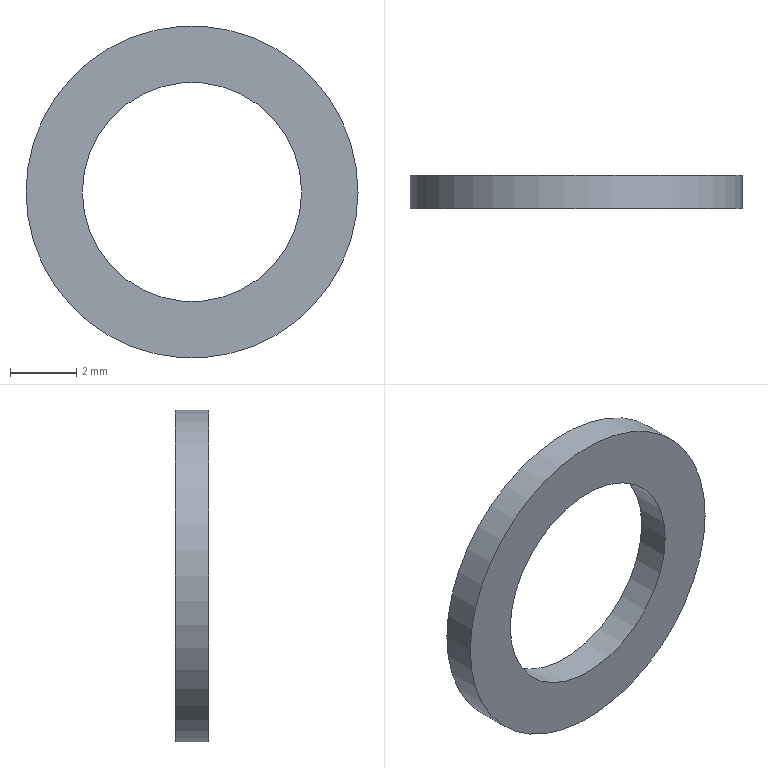Component | NX | WASHER_6_2 | 1 solid | 4 faces | box 10 x 1 x 10 mm | volume 44 mm3 | cylinder 2 | plane 2 | commonest cylinder face diameters 10 x1 6.6 x1
STEP:
#1=CARTESIAN_POINT('',(0.,0.,0.));
#2=DIRECTION('',(0.,0.,1.));
#3=DIRECTION('',(1.,0.,0.));
#4=AXIS2_PLACEMENT_3D('',#1,#2,#3);
#5=CARTESIAN_POINT('',(35.,2.,-0.));
#6=VERTEX_POINT('',#5);
#7=CARTESIAN_POINT('',(30.,2.,0.));
#8=DIRECTION('',(0.,-1.,0.));
#9=DIRECTION('',(1.,0.,-0.));
#10=AXIS2_PLACEMENT_3D('',#7,#8,#9);
#11=CIRCLE('',#10,5.);
#12=CARTESIAN_POINT('',(30.,2.,0.));
#13=DIRECTION('',(0.,1.,0.));
#14=DIRECTION('',(0.,0.,1.));
#15=AXIS2_PLACEMENT_3D('',#12,#13,#14);
#16=CYLINDRICAL_SURFACE('',#15,5.);
#17=CARTESIAN_POINT('',(7.854,0.));
#18=DIRECTION('',(-1.,0.));
#19=VECTOR('',#18,1.);
#20=LINE('',#17,#19);
#21=(GEOMETRIC_REPRESENTATION_CONTEXT(2)PARAMETRIC_REPRESENTATION_CONTEXT()REPRESENTATION_CONTEXT('',''));
#22=DEFINITIONAL_REPRESENTATION('',(#20),#21);
#23=PCURVE('',#16,#22);
#24=CARTESIAN_POINT('',(30.,2.,0.));
#25=DIRECTION('',(0.,-1.,0.));
#26=DIRECTION('',(0.,0.,-1.));
#27=AXIS2_PLACEMENT_3D('',#24,#25,#26);
#28=PLANE('',#27);
#29=CARTESIAN_POINT('',(0.,0.));
#30=DIRECTION('',(0.,1.));
#31=AXIS2_PLACEMENT_2D('',#29,#30);
#32=CIRCLE('',#31,5.);
#33=(GEOMETRIC_REPRESENTATION_CONTEXT(2)PARAMETRIC_REPRESENTATION_CONTEXT()REPRESENTATION_CONTEXT('',''));
#34=DEFINITIONAL_REPRESENTATION('',(#32),#33);
#35=PCURVE('',#28,#34);
#36=SURFACE_CURVE('',#11,(#23,#35),.PCURVE_S1.);
#37=EDGE_CURVE('',#6,#6,#36,.T.);
#38=ORIENTED_EDGE('',*,*,#37,.F.);
#39=CARTESIAN_POINT('',(35.,3.,-0.));
#40=VERTEX_POINT('',#39);
#41=CARTESIAN_POINT('',(35.,2.,0.));
#42=CARTESIAN_POINT('',(35.,3.,0.));
#43=B_SPLINE_CURVE_WITH_KNOTS('',1,(#41,#42),.UNSPECIFIED.,.F.,.F.,(2,2),(0.,1.),.PIECEWISE_BEZIER_KNOTS.);
#44=CARTESIAN_POINT('',(7.854,0.));
#45=DIRECTION('',(0.,1.));
#46=VECTOR('',#45,1.);
#47=LINE('',#44,#46);
#48=(GEOMETRIC_REPRESENTATION_CONTEXT(2)PARAMETRIC_REPRESENTATION_CONTEXT()REPRESENTATION_CONTEXT('',''));
#49=DEFINITIONAL_REPRESENTATION('',(#47),#48);
#50=PCURVE('',#16,#49);
#51=CARTESIAN_POINT('',(1.571,0.));
#52=DIRECTION('',(0.,1.));
#53=VECTOR('',#52,1.);
#54=LINE('',#51,#53);
#55=(GEOMETRIC_REPRESENTATION_CONTEXT(2)PARAMETRIC_REPRESENTATION_CONTEXT()REPRESENTATION_CONTEXT('',''));
#56=DEFINITIONAL_REPRESENTATION('',(#54),#55);
#57=PCURVE('',#16,#56);
#58=SEAM_CURVE('',#43,(#50,#57),.PCURVE_S1.);
#59=EDGE_CURVE('',#6,#40,#58,.T.);
#60=ORIENTED_EDGE('',*,*,#59,.T.);
#61=CARTESIAN_POINT('',(30.,3.,0.));
#62=DIRECTION('',(0.,-1.,0.));
#63=DIRECTION('',(1.,0.,-0.));
#64=AXIS2_PLACEMENT_3D('',#61,#62,#63);
#65=CIRCLE('',#64,5.);
#66=CARTESIAN_POINT('',(7.854,1.));
#67=DIRECTION('',(-1.,0.));
#68=VECTOR('',#67,1.);
#69=LINE('',#66,#68);
#70=(GEOMETRIC_REPRESENTATION_CONTEXT(2)PARAMETRIC_REPRESENTATION_CONTEXT()REPRESENTATION_CONTEXT('',''));
#71=DEFINITIONAL_REPRESENTATION('',(#69),#70);
#72=PCURVE('',#16,#71);
#73=CARTESIAN_POINT('',(30.,3.,0.));
#74=DIRECTION('',(0.,-1.,0.));
#75=DIRECTION('',(0.,0.,-1.));
#76=AXIS2_PLACEMENT_3D('',#73,#74,#75);
#77=PLANE('',#76);
#78=CARTESIAN_POINT('',(0.,0.));
#79=DIRECTION('',(0.,1.));
#80=AXIS2_PLACEMENT_2D('',#78,#79);
#81=CIRCLE('',#80,5.);
#82=(GEOMETRIC_REPRESENTATION_CONTEXT(2)PARAMETRIC_REPRESENTATION_CONTEXT()REPRESENTATION_CONTEXT('',''));
#83=DEFINITIONAL_REPRESENTATION('',(#81),#82);
#84=PCURVE('',#77,#83);
#85=SURFACE_CURVE('',#65,(#72,#84),.PCURVE_S1.);
#86=EDGE_CURVE('',#40,#40,#85,.T.);
#87=ORIENTED_EDGE('',*,*,#86,.T.);
#88=ORIENTED_EDGE('',*,*,#59,.F.);
#89=EDGE_LOOP('',(#38,#60,#87,#88));
#90=FACE_BOUND('',#89,.T.);
#91=ADVANCED_FACE('',(#90),#16,.T.);
#92=CARTESIAN_POINT('',(33.3,2.,-0.));
#93=VERTEX_POINT('',#92);
#94=CARTESIAN_POINT('',(30.,2.,0.));
#95=DIRECTION('',(0.,-1.,0.));
#96=DIRECTION('',(1.,0.,-0.));
#97=AXIS2_PLACEMENT_3D('',#94,#95,#96);
#98=CIRCLE('',#97,3.3);
#99=CARTESIAN_POINT('',(30.,2.,0.));
#100=DIRECTION('',(0.,1.,0.));
#101=DIRECTION('',(0.,0.,1.));
#102=AXIS2_PLACEMENT_3D('',#99,#100,#101);
#103=CYLINDRICAL_SURFACE('',#102,3.3);
#104=CARTESIAN_POINT('',(7.854,0.));
#105=DIRECTION('',(-1.,0.));
#106=VECTOR('',#105,1.);
#107=LINE('',#104,#106);
#108=(GEOMETRIC_REPRESENTATION_CONTEXT(2)PARAMETRIC_REPRESENTATION_CONTEXT()REPRESENTATION_CONTEXT('',''));
#109=DEFINITIONAL_REPRESENTATION('',(#107),#108);
#110=PCURVE('',#103,#109);
#111=CARTESIAN_POINT('',(0.,0.));
#112=DIRECTION('',(0.,1.));
#113=AXIS2_PLACEMENT_2D('',#111,#112);
#114=CIRCLE('',#113,3.3);
#115=(GEOMETRIC_REPRESENTATION_CONTEXT(2)PARAMETRIC_REPRESENTATION_CONTEXT()REPRESENTATION_CONTEXT('',''));
#116=DEFINITIONAL_REPRESENTATION('',(#114),#115);
#117=PCURVE('',#28,#116);
#118=SURFACE_CURVE('',#98,(#110,#117),.PCURVE_S1.);
#119=EDGE_CURVE('',#93,#93,#118,.T.);
#120=ORIENTED_EDGE('',*,*,#119,.F.);
#121=CARTESIAN_POINT('',(33.3,3.,-0.));
#122=VERTEX_POINT('',#121);
#123=CARTESIAN_POINT('',(33.3,2.,0.));
#124=CARTESIAN_POINT('',(33.3,3.,0.));
#125=B_SPLINE_CURVE_WITH_KNOTS('',1,(#123,#124),.UNSPECIFIED.,.F.,.F.,(2,2),(0.,1.),.PIECEWISE_BEZIER_KNOTS.);
#126=CARTESIAN_POINT('',(7.854,0.));
#127=DIRECTION('',(0.,1.));
#128=VECTOR('',#127,1.);
#129=LINE('',#126,#128);
#130=(GEOMETRIC_REPRESENTATION_CONTEXT(2)PARAMETRIC_REPRESENTATION_CONTEXT()REPRESENTATION_CONTEXT('',''));
#131=DEFINITIONAL_REPRESENTATION('',(#129),#130);
#132=PCURVE('',#103,#131);
#133=CARTESIAN_POINT('',(1.571,0.));
#134=DIRECTION('',(0.,1.));
#135=VECTOR('',#134,1.);
#136=LINE('',#133,#135);
#137=(GEOMETRIC_REPRESENTATION_CONTEXT(2)PARAMETRIC_REPRESENTATION_CONTEXT()REPRESENTATION_CONTEXT('',''));
#138=DEFINITIONAL_REPRESENTATION('',(#136),#137);
#139=PCURVE('',#103,#138);
#140=SEAM_CURVE('',#125,(#132,#139),.PCURVE_S1.);
#141=EDGE_CURVE('',#93,#122,#140,.T.);
#142=ORIENTED_EDGE('',*,*,#141,.T.);
#143=CARTESIAN_POINT('',(30.,3.,0.));
#144=DIRECTION('',(0.,-1.,0.));
#145=DIRECTION('',(1.,0.,-0.));
#146=AXIS2_PLACEMENT_3D('',#143,#144,#145);
#147=CIRCLE('',#146,3.3);
#148=CARTESIAN_POINT('',(7.854,1.));
#149=DIRECTION('',(-1.,0.));
#150=VECTOR('',#149,1.);
#151=LINE('',#148,#150);
#152=(GEOMETRIC_REPRESENTATION_CONTEXT(2)PARAMETRIC_REPRESENTATION_CONTEXT()REPRESENTATION_CONTEXT('',''));
#153=DEFINITIONAL_REPRESENTATION('',(#151),#152);
#154=PCURVE('',#103,#153);
#155=CARTESIAN_POINT('',(0.,0.));
#156=DIRECTION('',(0.,1.));
#157=AXIS2_PLACEMENT_2D('',#155,#156);
#158=CIRCLE('',#157,3.3);
#159=(GEOMETRIC_REPRESENTATION_CONTEXT(2)PARAMETRIC_REPRESENTATION_CONTEXT()REPRESENTATION_CONTEXT('',''));
#160=DEFINITIONAL_REPRESENTATION('',(#158),#159);
#161=PCURVE('',#77,#160);
#162=SURFACE_CURVE('',#147,(#154,#161),.PCURVE_S1.);
#163=EDGE_CURVE('',#122,#122,#162,.T.);
#164=ORIENTED_EDGE('',*,*,#163,.T.);
#165=ORIENTED_EDGE('',*,*,#141,.F.);
#166=EDGE_LOOP('',(#120,#142,#164,#165));
#167=FACE_BOUND('',#166,.F.);
#168=ADVANCED_FACE('',(#167),#103,.F.);
#169=ORIENTED_EDGE('',*,*,#37,.T.);
#170=EDGE_LOOP('',(#169));
#171=FACE_BOUND('',#170,.T.);
#172=ORIENTED_EDGE('',*,*,#119,.F.);
#173=EDGE_LOOP('',(#172));
#174=FACE_BOUND('',#173,.T.);
#175=ADVANCED_FACE('',(#171,#174),#28,.T.);
#176=ORIENTED_EDGE('',*,*,#86,.F.);
#177=EDGE_LOOP('',(#176));
#178=FACE_BOUND('',#177,.T.);
#179=ORIENTED_EDGE('',*,*,#163,.T.);
#180=EDGE_LOOP('',(#179));
#181=FACE_BOUND('',#180,.T.);
#182=ADVANCED_FACE('',(#178,#181),#77,.F.);
#183=CLOSED_SHELL('',(#91,#168,#175,#182));
#184=MANIFOLD_SOLID_BREP('',#183);
#185=(LENGTH_UNIT()NAMED_UNIT(*)SI_UNIT(.MILLI.,.METRE.));
#186=UNCERTAINTY_MEASURE_WITH_UNIT(LENGTH_MEASURE(0.00001),#185,'','');
#187=(NAMED_UNIT(*)PLANE_ANGLE_UNIT()SI_UNIT($,.RADIAN.));
#188=(NAMED_UNIT(*)SI_UNIT($,.STERADIAN.)SOLID_ANGLE_UNIT());
#189=(GEOMETRIC_REPRESENTATION_CONTEXT(3)GLOBAL_UNCERTAINTY_ASSIGNED_CONTEXT((#186))GLOBAL_UNIT_ASSIGNED_CONTEXT((#185,#187,#188))REPRESENTATION_CONTEXT('',''));
#190=ADVANCED_BREP_SHAPE_REPRESENTATION('',(#4,#184),#189);